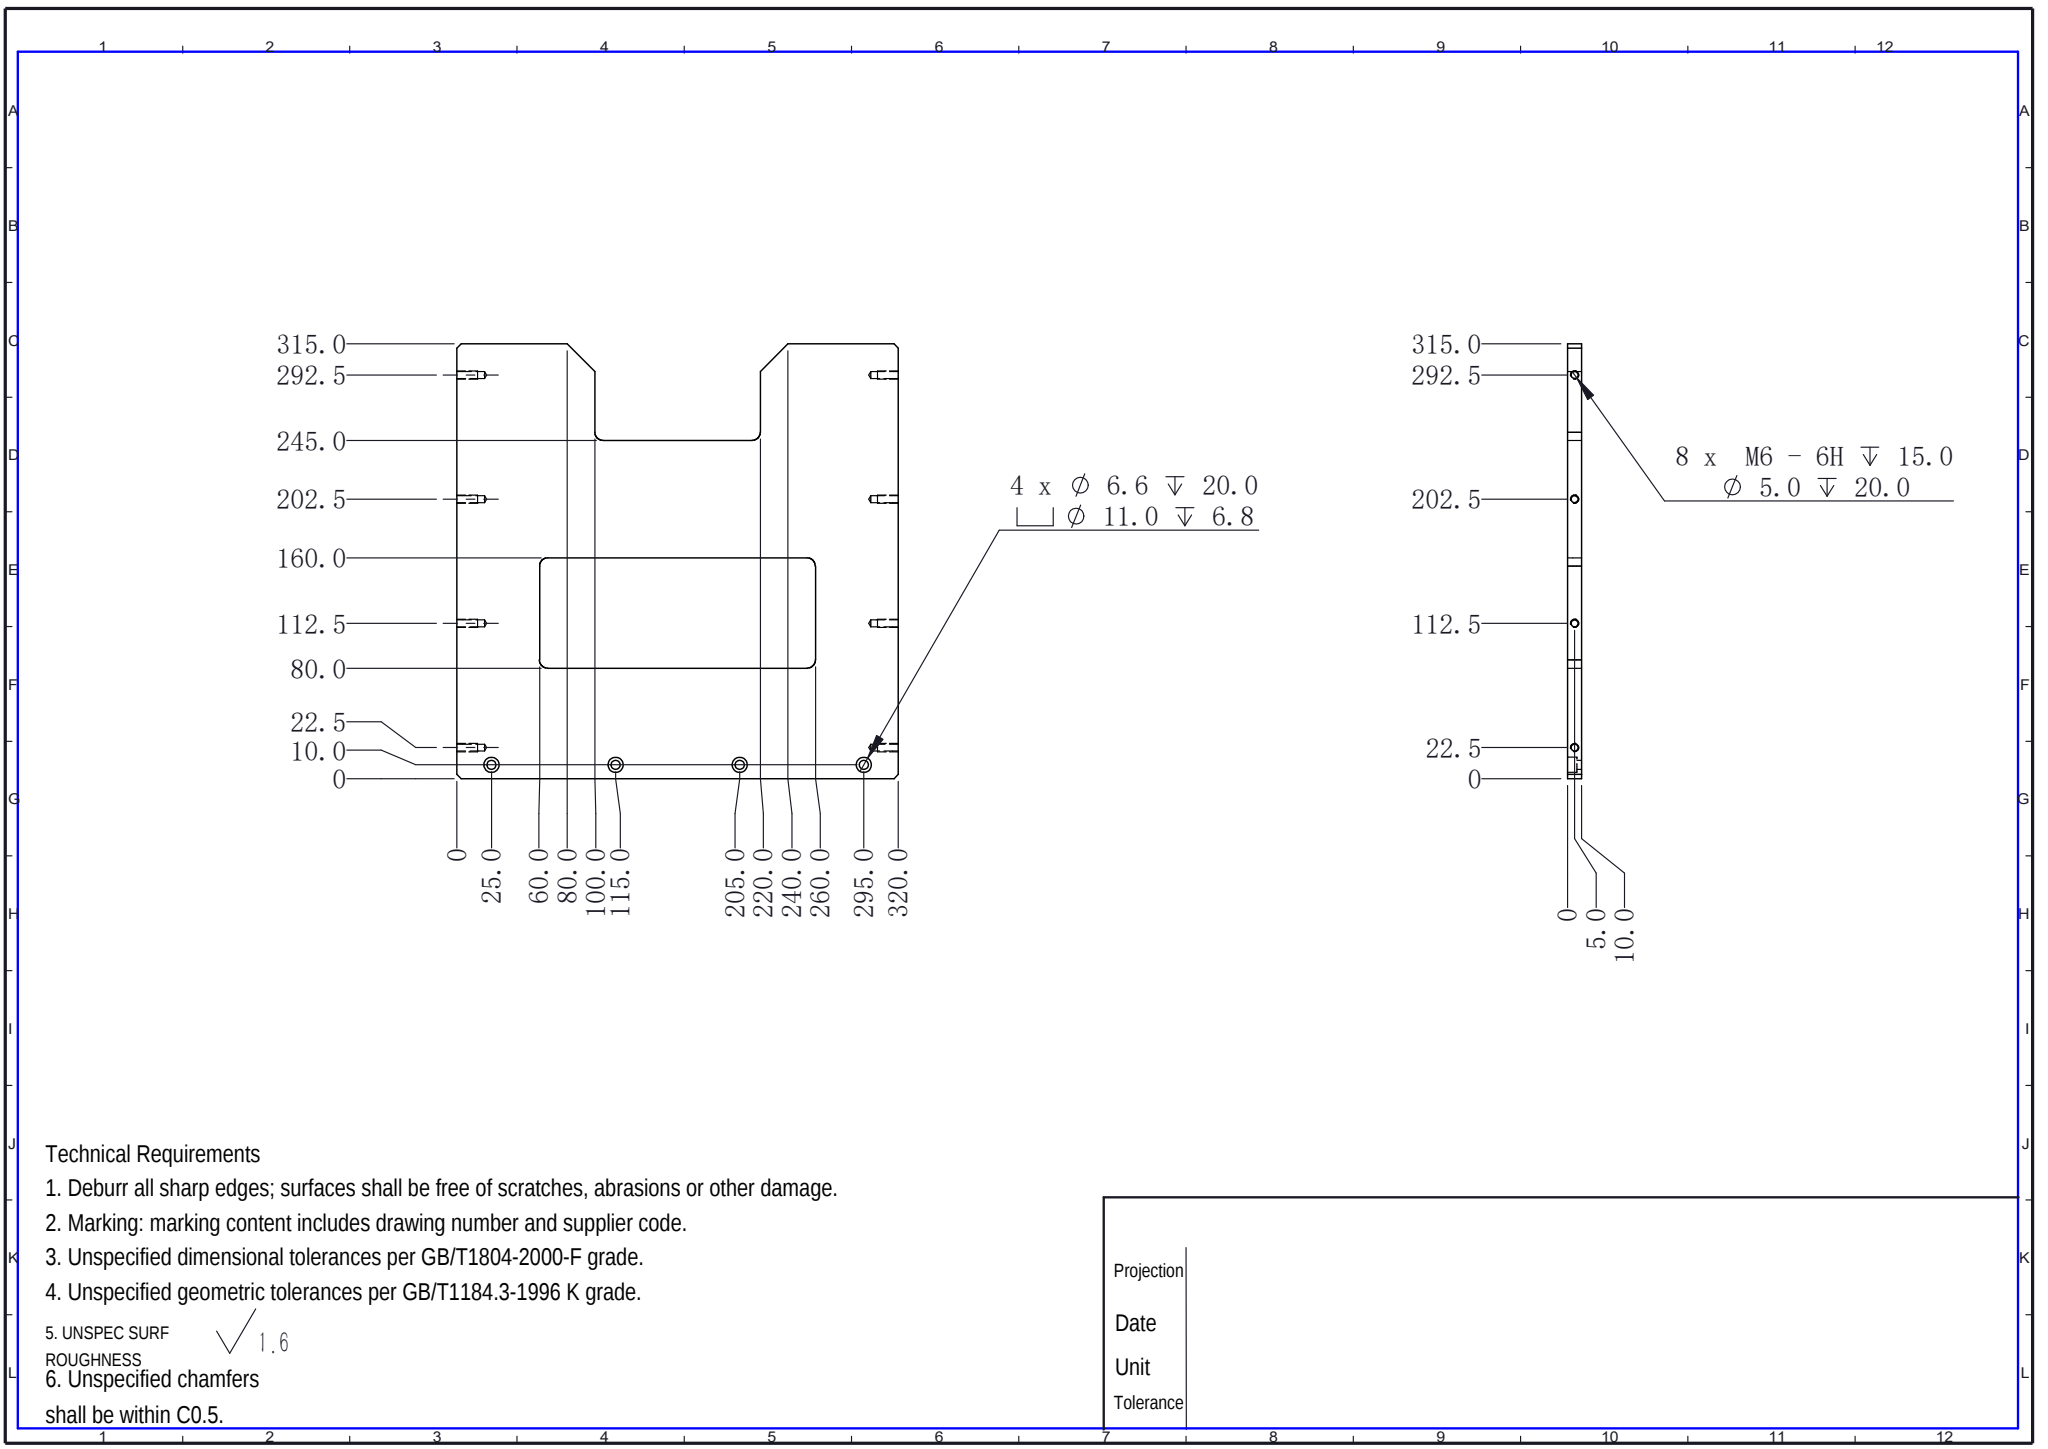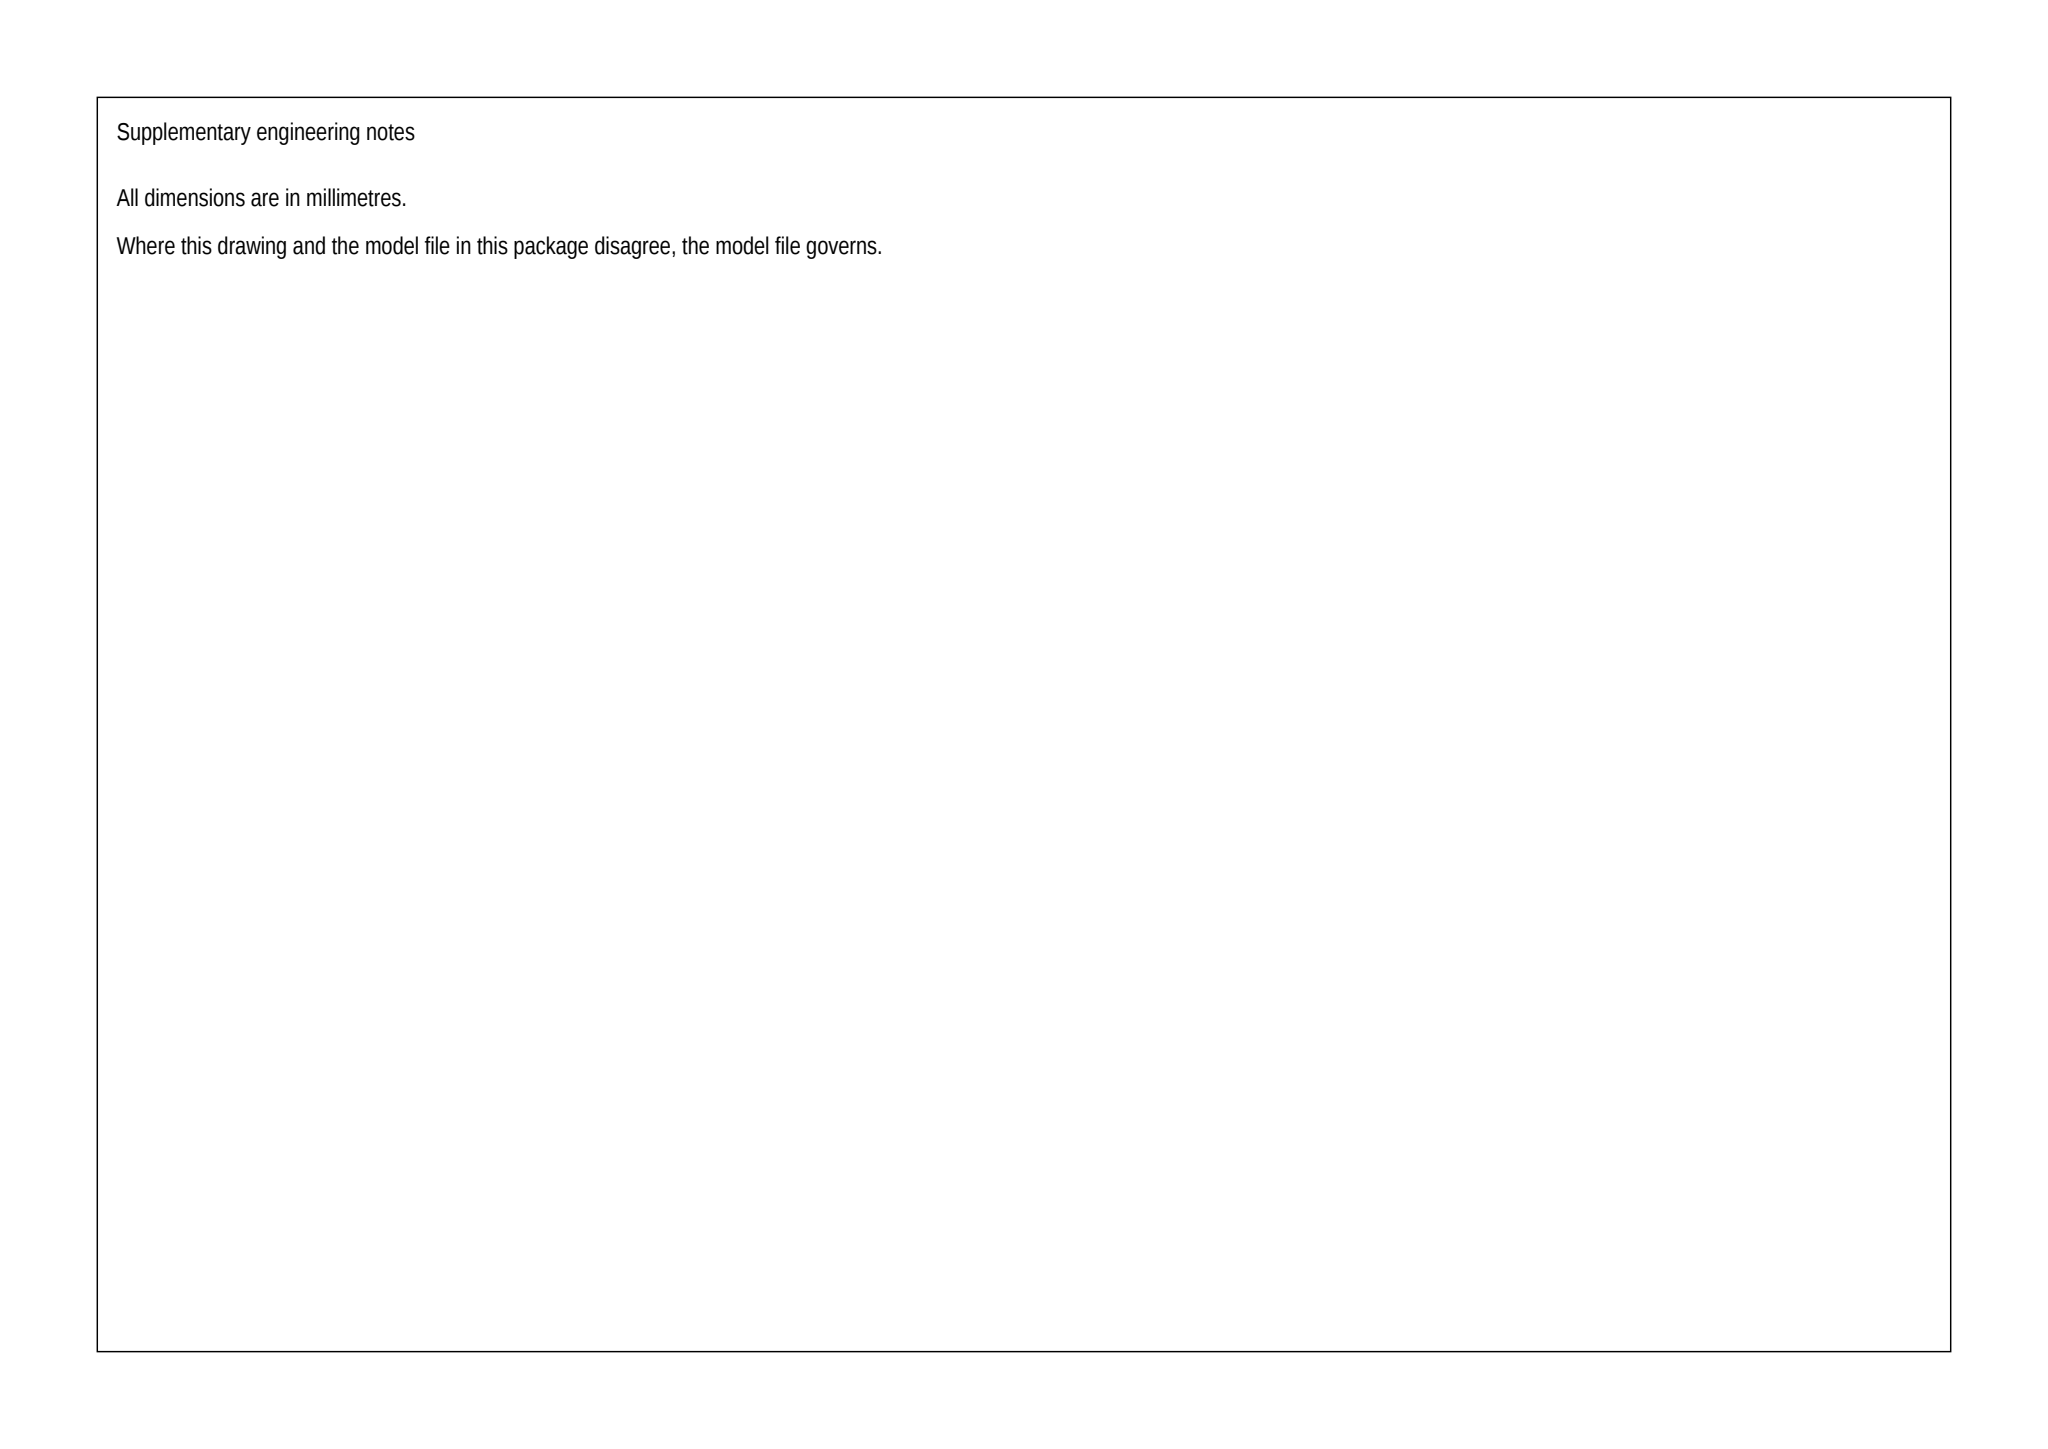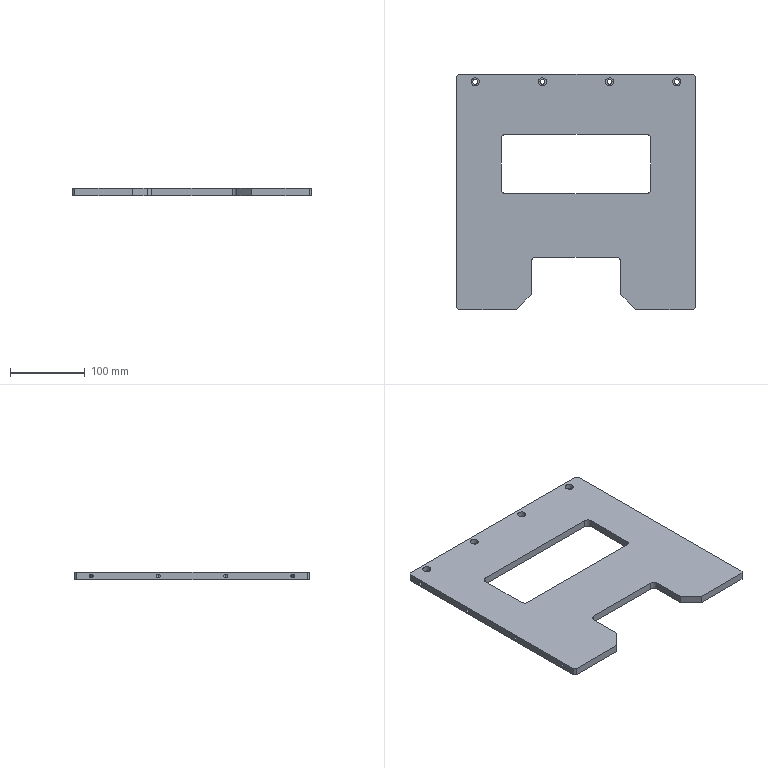Part | SolidWorks | mm | 1 solid | 78 faces | box 320 x 315 x 10 mm | volume 754040 mm3 | cylinder 38 | plane 24 | cone 16 | commonest cylinder face diameters 5 x16 11 x8 6.6 x8 12 x6
Drawing notes:
CENTRAL CUTOUT 200 x 80 THRU, R6 CORNERS; X 60-260, Y 80-160 | from the solid: Planes x=60/260 and y=155/235 (=Y 80-160) with Ø12 thru cyls (len 10) at (66,161),(66,229),(254,161),(254,229) -> R6 corners
R6 AT TOP NOTCH INNER CORNERS, X 100 & X 220 AT Y 245, THRU | from the solid: Ø12 z-axis cyls len 10 (full thk) at (106,64) and (214,64), 6 mm inside planes x=100/220 and y=70 (=Y 245)
build123d program:
from build123d import *

# Parameters (mm, degrees)
SKETCH1_W                                           = 200
SKETCH1_H                                           = 80
BOSS_EXTRUDE1_DEPTH                                 = 5
M6_TAPPED_HOLE1_AT_2_COUNT                          = 2
M6_TAPPED_HOLE1_AT_2_PITCH                          = 90
M6_TAPPED_HOLE1_AT_3_COUNT                          = 2
M6_TAPPED_HOLE1_AT_3_PITCH                          = 180
M6_TAPPED_HOLE1_AT_4_COUNT                          = 2
M6_TAPPED_HOLE1_AT_4_PITCH                          = 270
HOLE_SIZE_ACCORDING_TO_TYPE_1_OF_HEXAGO_D           = 6.6
HOLE_SIZE_ACCORDING_TO_TYPE_1_OF_HEXAGO_DEPTH       = 20
HOLE_SIZE_ACCORDING_TO_TYPE_1_OF_HEXAGO_CBORE_D     = 11
HOLE_SIZE_ACCORDING_TO_TYPE_1_OF_HEXAGO_CBORE_DEPTH = 6.8
HOLE_SIZE_ACCORDING_TO_TYPE_1_OF_HEXAGO_TIP         = 1.983
FILLET1_R                                           = 6
CHAMFER1_SIZE                                       = 20
CHAMFER2_SIZE                                       = 3


with BuildPart() as part:
    # Sketch1 → Boss-Extrude1 (new, symmetric)
    with BuildSketch(Plane.XY):
        Polygon((-160, 157.5), (160, 157.5), (160, -157.5), (60, -157.5), (60, -87.5), (-60, -87.5), (-60, -157.5), (-160, -157.5), align=None)
        with Locations((0, 37.5)):
            Rectangle(SKETCH1_W, SKETCH1_H, mode=Mode.SUBTRACT)
    extrude(amount=BOSS_EXTRUDE1_DEPTH, both=True)

    # Sketch3 → M6 Tapped Hole1 (revolve, cut)
    with BuildSketch(Plane(origin=(-160, 135, 0), x_dir=(0, 0, 1), z_dir=(0, 1, 0))):
        Polygon((0, 0), (0, 21.502), (2.5, 20), (2.5, 0), align=None)
    m6_tapped_hole1 = revolve(axis=Axis((-166.35, 135, 0), (1, 0, 0)), mode=Mode.SUBTRACT)

    # M6 Tapped Hole1 at 2: M6 Tapped Hole1 ×2
    with Locations(*[(0, -i * M6_TAPPED_HOLE1_AT_2_PITCH, 0) for i in range(1, M6_TAPPED_HOLE1_AT_2_COUNT)]):
        add(m6_tapped_hole1, mode=Mode.SUBTRACT)

    # M6 Tapped Hole1 at 3: M6 Tapped Hole1 ×2
    with Locations(*[(0, -i * M6_TAPPED_HOLE1_AT_3_PITCH, 0) for i in range(1, M6_TAPPED_HOLE1_AT_3_COUNT)]):
        add(m6_tapped_hole1, mode=Mode.SUBTRACT)

    # M6 Tapped Hole1 at 4: M6 Tapped Hole1 ×2
    with Locations(*[(0, -i * M6_TAPPED_HOLE1_AT_4_PITCH, 0) for i in range(1, M6_TAPPED_HOLE1_AT_4_COUNT)]):
        add(m6_tapped_hole1, mode=Mode.SUBTRACT)

    # Mirror1: M6 Tapped Hole1 across plane
    add(m6_tapped_hole1.mirror(Plane(origin=(0, 0, 0), x_dir=(0, 0, 1), z_dir=(1, 0, 0))), mode=Mode.SUBTRACT)

    # Mirror1 copy 1 sketch → Mirror1 copy 1 (revolve, cut)
    with BuildSketch(Plane(origin=(160, 45, 0), x_dir=(0, 0, 1), z_dir=(0, 1, 0))):
        Polygon((0, 0), (0, -21.502), (2.5, -20), (2.5, 0), align=None)
    revolve(axis=Axis((166.35, 45, 0), (1, 0, 0)), mode=Mode.SUBTRACT)

    # Mirror1 copy 2 sketch → Mirror1 copy 2 (revolve, cut)
    with BuildSketch(Plane(origin=(160, -45, 0), x_dir=(0, 0, 1), z_dir=(0, 1, 0))):
        Polygon((0, 0), (0, -21.502), (2.5, -20), (2.5, 0), align=None)
    revolve(axis=Axis((166.35, -45, 0), (1, 0, 0)), mode=Mode.SUBTRACT)

    # Mirror1 copy 3 sketch → Mirror1 copy 3 (revolve, cut)
    with BuildSketch(Plane(origin=(160, -135, 0), x_dir=(0, 0, 1), z_dir=(0, 1, 0))):
        Polygon((0, 0), (0, -21.502), (2.5, -20), (2.5, 0), align=None)
    revolve(axis=Axis((166.35, -135, 0), (1, 0, 0)), mode=Mode.SUBTRACT)

    # Hole Size_According to_ Type 1 of Hexago
    with Locations(Plane.XY.offset(5)):
        with Locations((135, 147.5), (45, 147.5), (-45, 147.5), (-135, 147.5)):
            CounterBoreHole(HOLE_SIZE_ACCORDING_TO_TYPE_1_OF_HEXAGO_D / 2, HOLE_SIZE_ACCORDING_TO_TYPE_1_OF_HEXAGO_CBORE_D / 2, HOLE_SIZE_ACCORDING_TO_TYPE_1_OF_HEXAGO_CBORE_DEPTH, depth=HOLE_SIZE_ACCORDING_TO_TYPE_1_OF_HEXAGO_DEPTH)
            with Locations((0, 0, -(HOLE_SIZE_ACCORDING_TO_TYPE_1_OF_HEXAGO_DEPTH + HOLE_SIZE_ACCORDING_TO_TYPE_1_OF_HEXAGO_TIP / 2))):  # 118° drill point
                Cone(0, HOLE_SIZE_ACCORDING_TO_TYPE_1_OF_HEXAGO_D / 2, HOLE_SIZE_ACCORDING_TO_TYPE_1_OF_HEXAGO_TIP, mode=Mode.SUBTRACT)

    # Fillet1
    fillet1_edges = [part.edges().sort_by_distance(p)[0] for p in [
        (60, -87.5, 0),
        (-60, -87.5, 0),
        (-100, 77.5, 0),
        (-100, -2.5, 0),
        (100, -2.5, 0),
        (100, 77.5, 0),
    ]]
    fillet(fillet1_edges, radius=FILLET1_R)

    # Chamfer1
    chamfer1_edges = [part.edges().sort_by_distance(p)[0] for p in [
        (60, -157.5, 0),
        (-60, -157.5, 0),
    ]]
    chamfer(chamfer1_edges, length=CHAMFER1_SIZE)

    # Chamfer2
    chamfer2_edges = [part.edges().sort_by_distance(p)[0] for p in [
        (-160, 157.5, 0),
        (160, 157.5, 0),
        (160, -157.5, 0),
        (-160, -157.5, 0),
    ]]
    chamfer(chamfer2_edges, length=CHAMFER2_SIZE)


solid = part.part